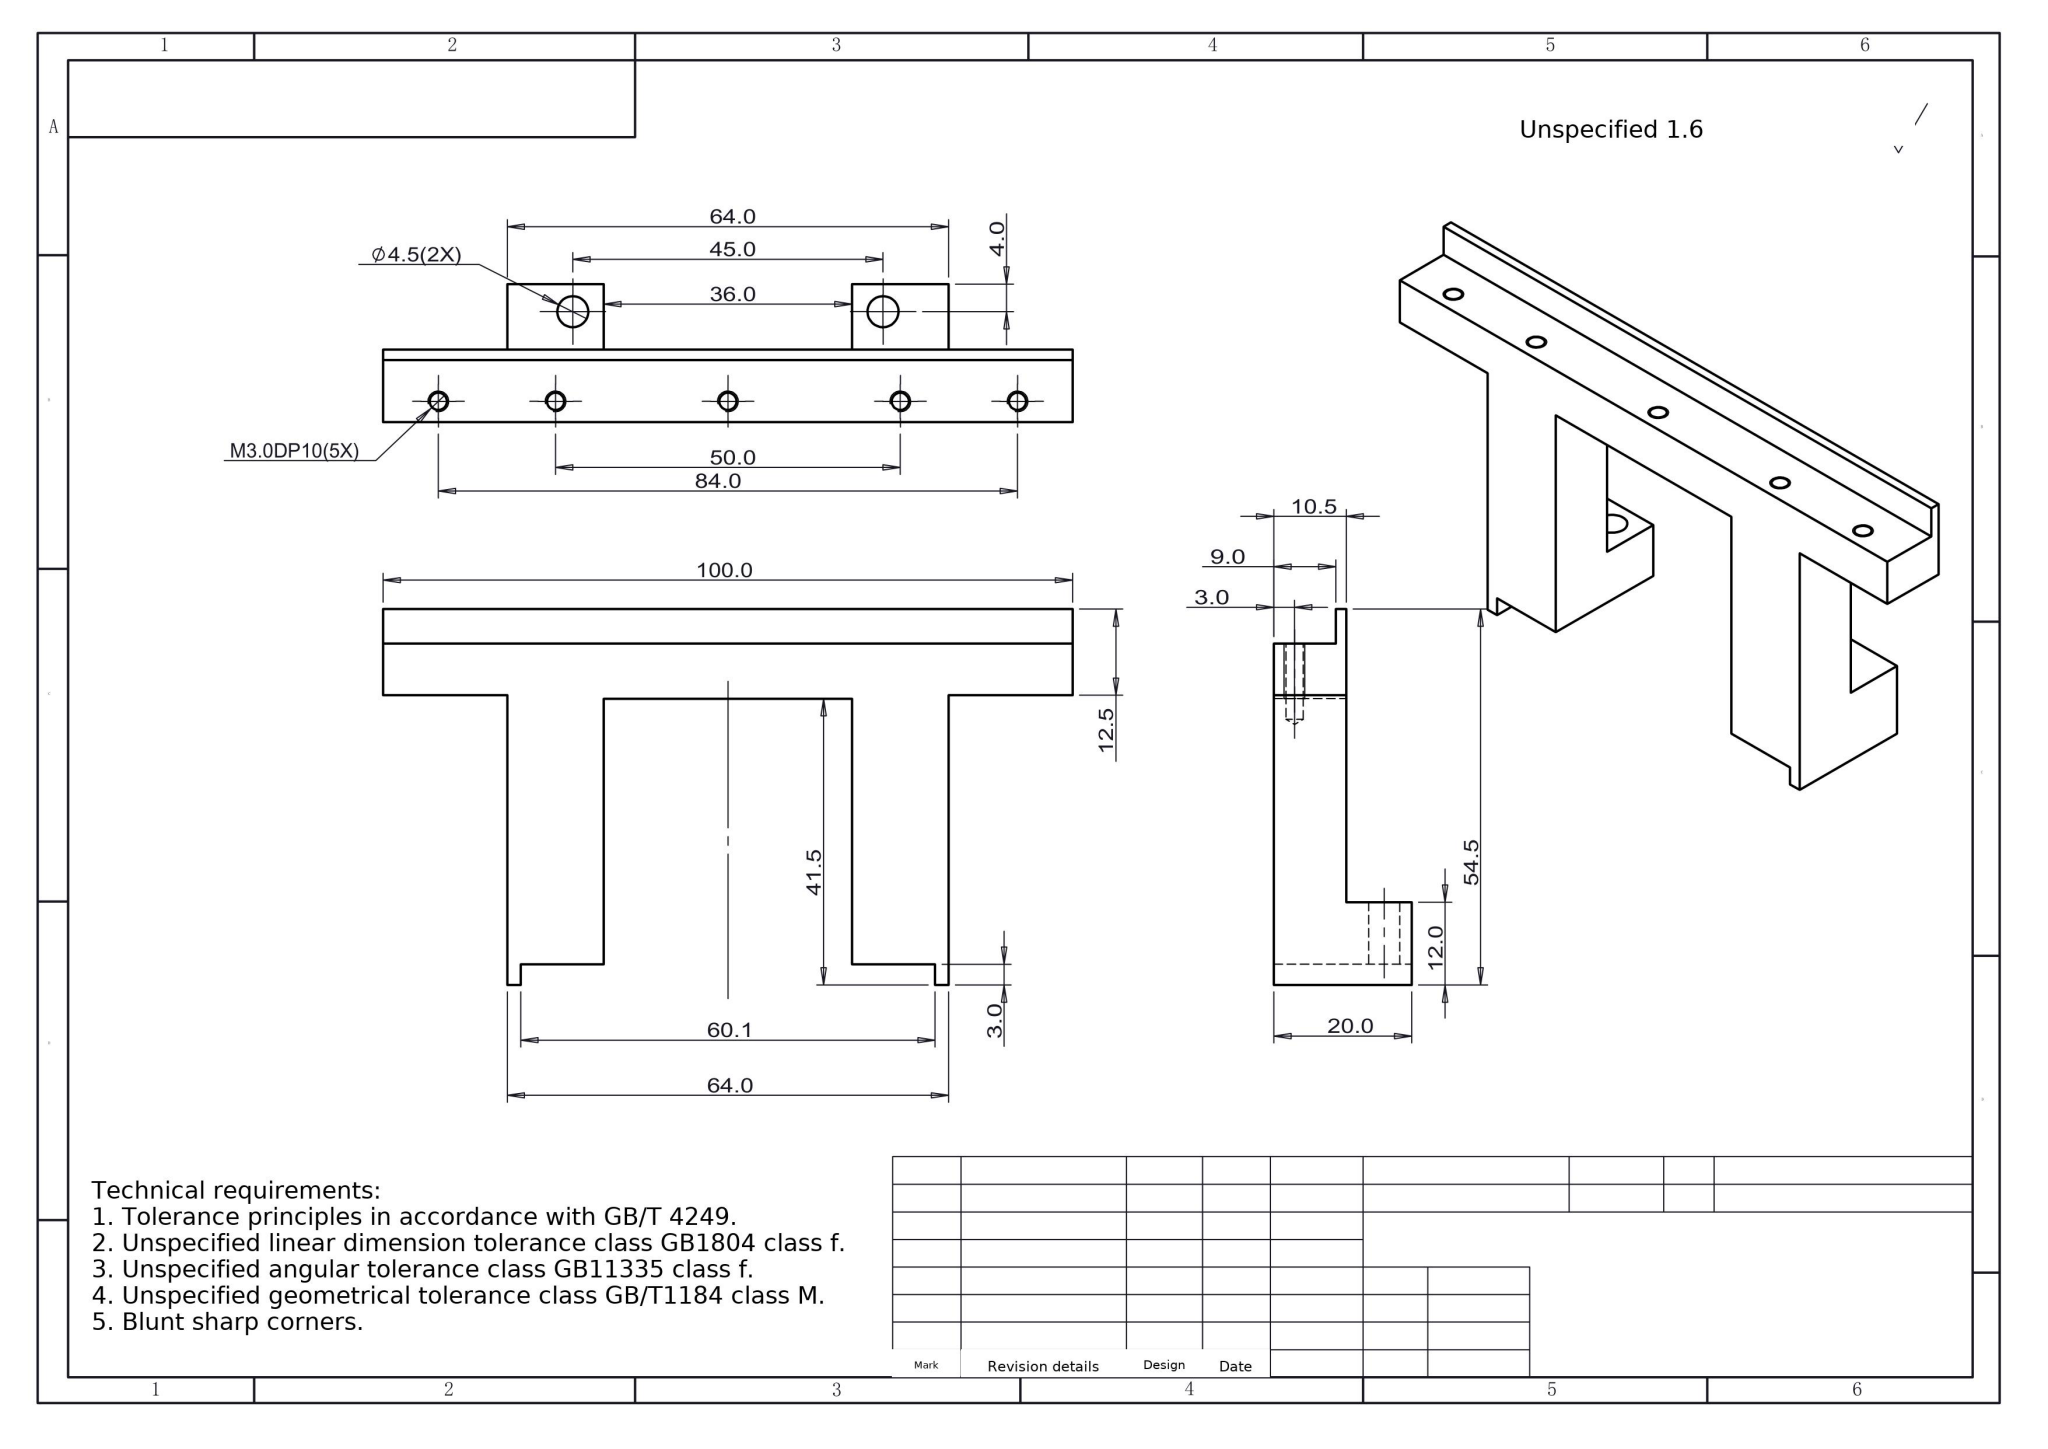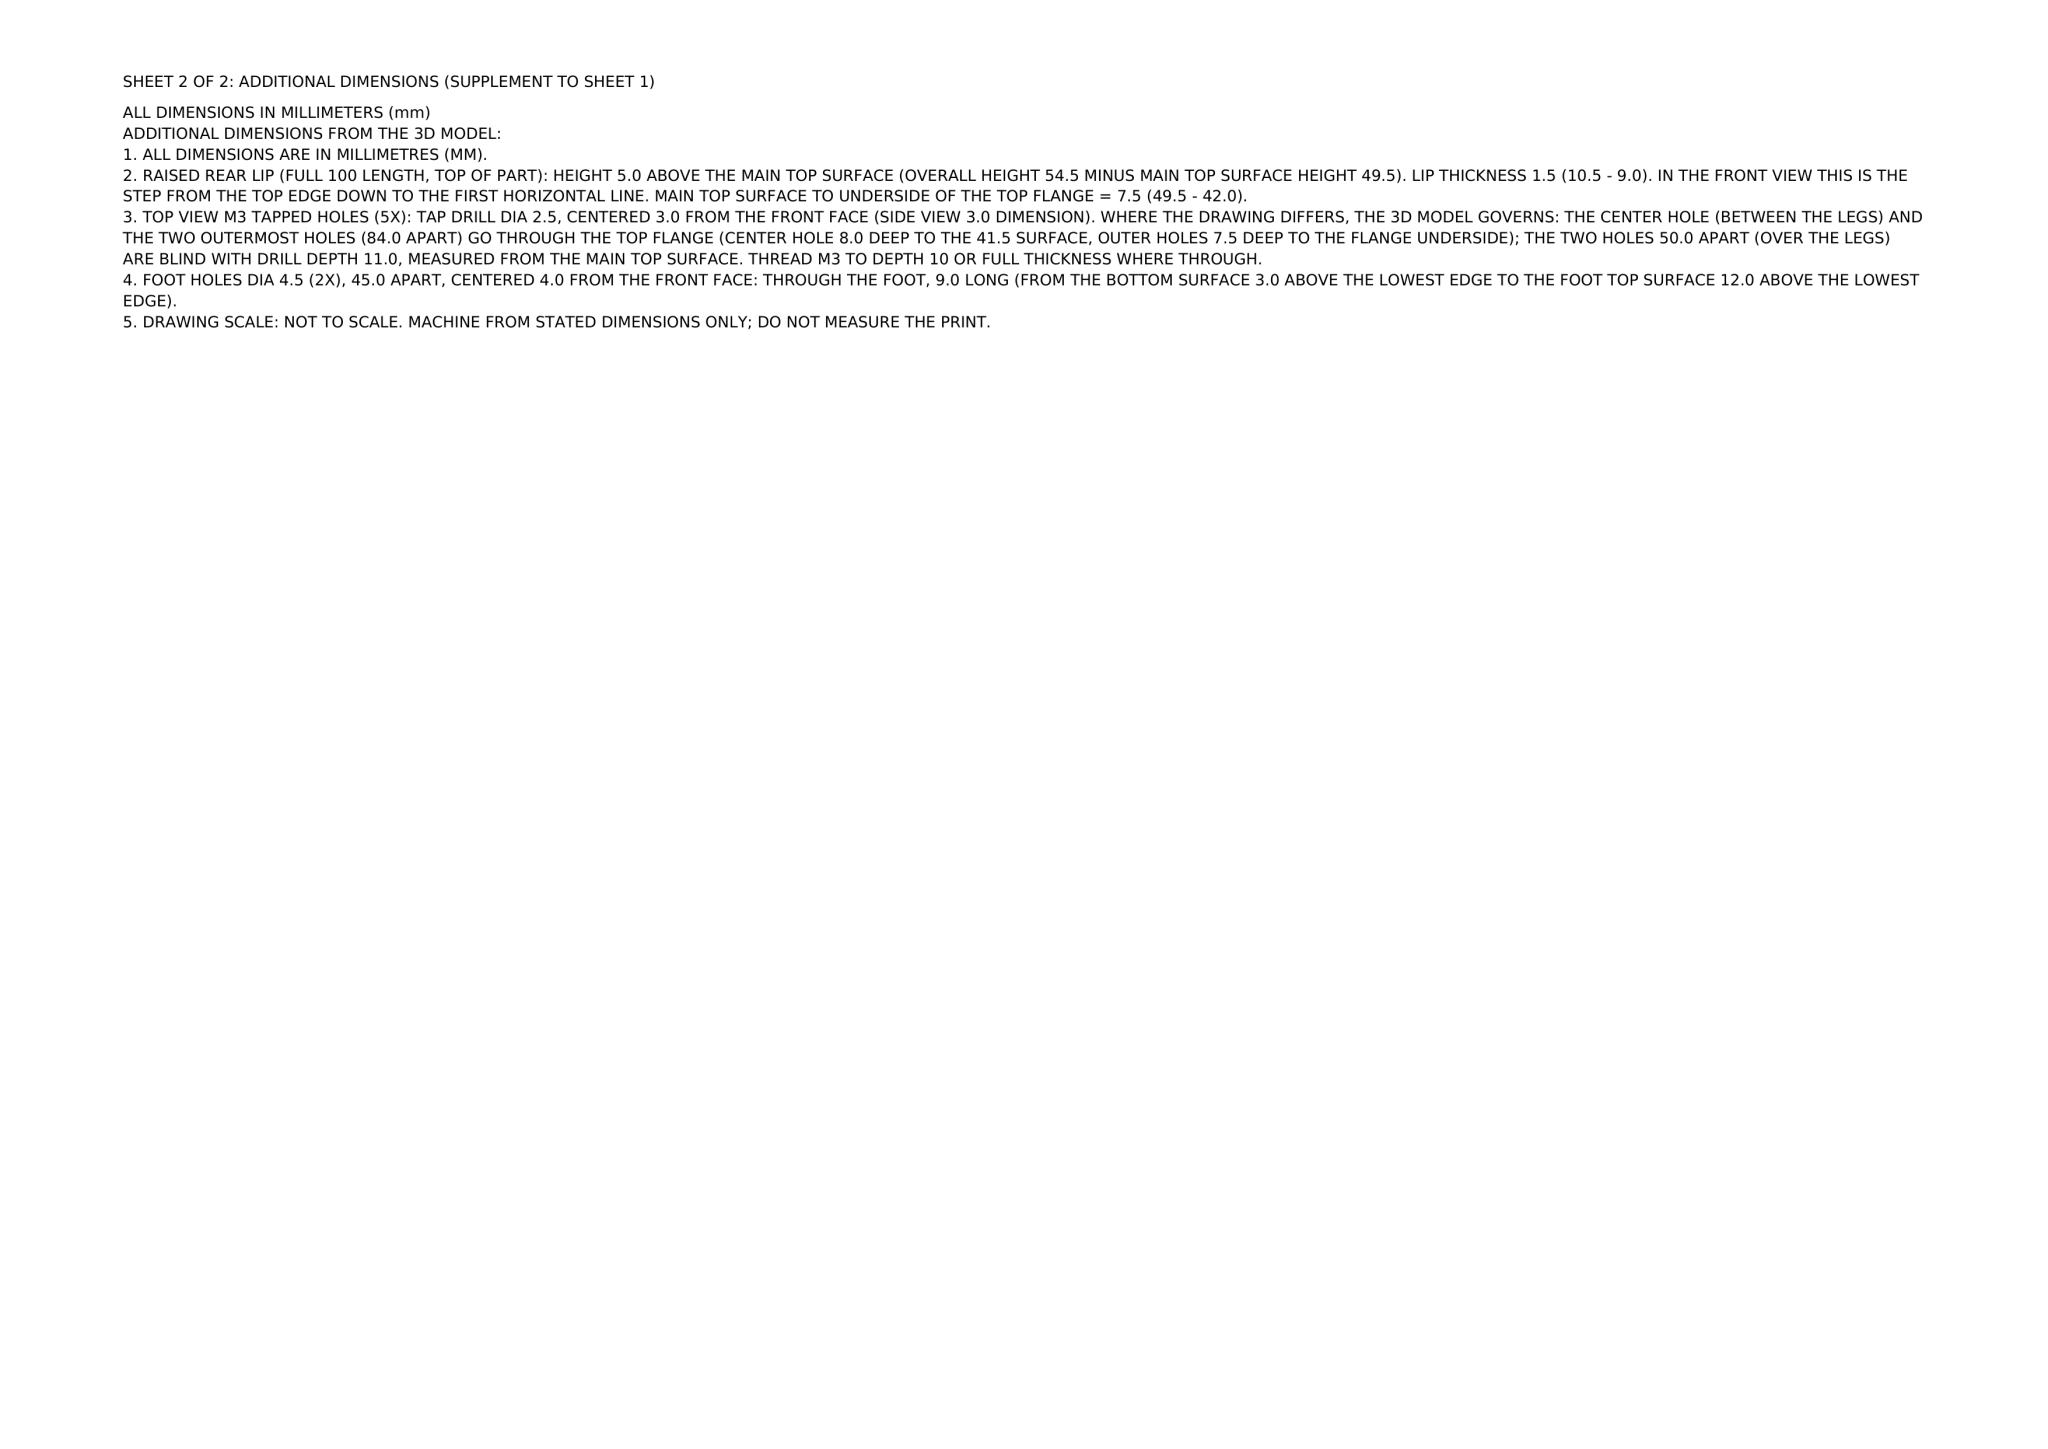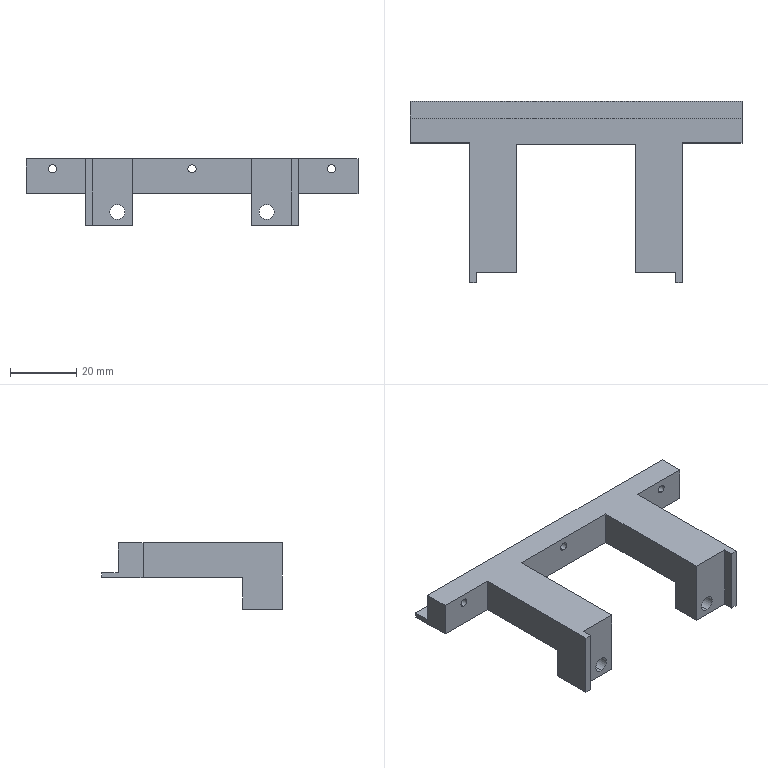Part | NX | mm | Dual U-Shaped Rail Bracket | 1 solid | 42 faces | box 100 x 54.5 x 20 mm | volume 22398 mm3 | plane 24 | cylinder 14 | cone 4 | commonest cylinder face diameters 2.5 x10 4.5 x4